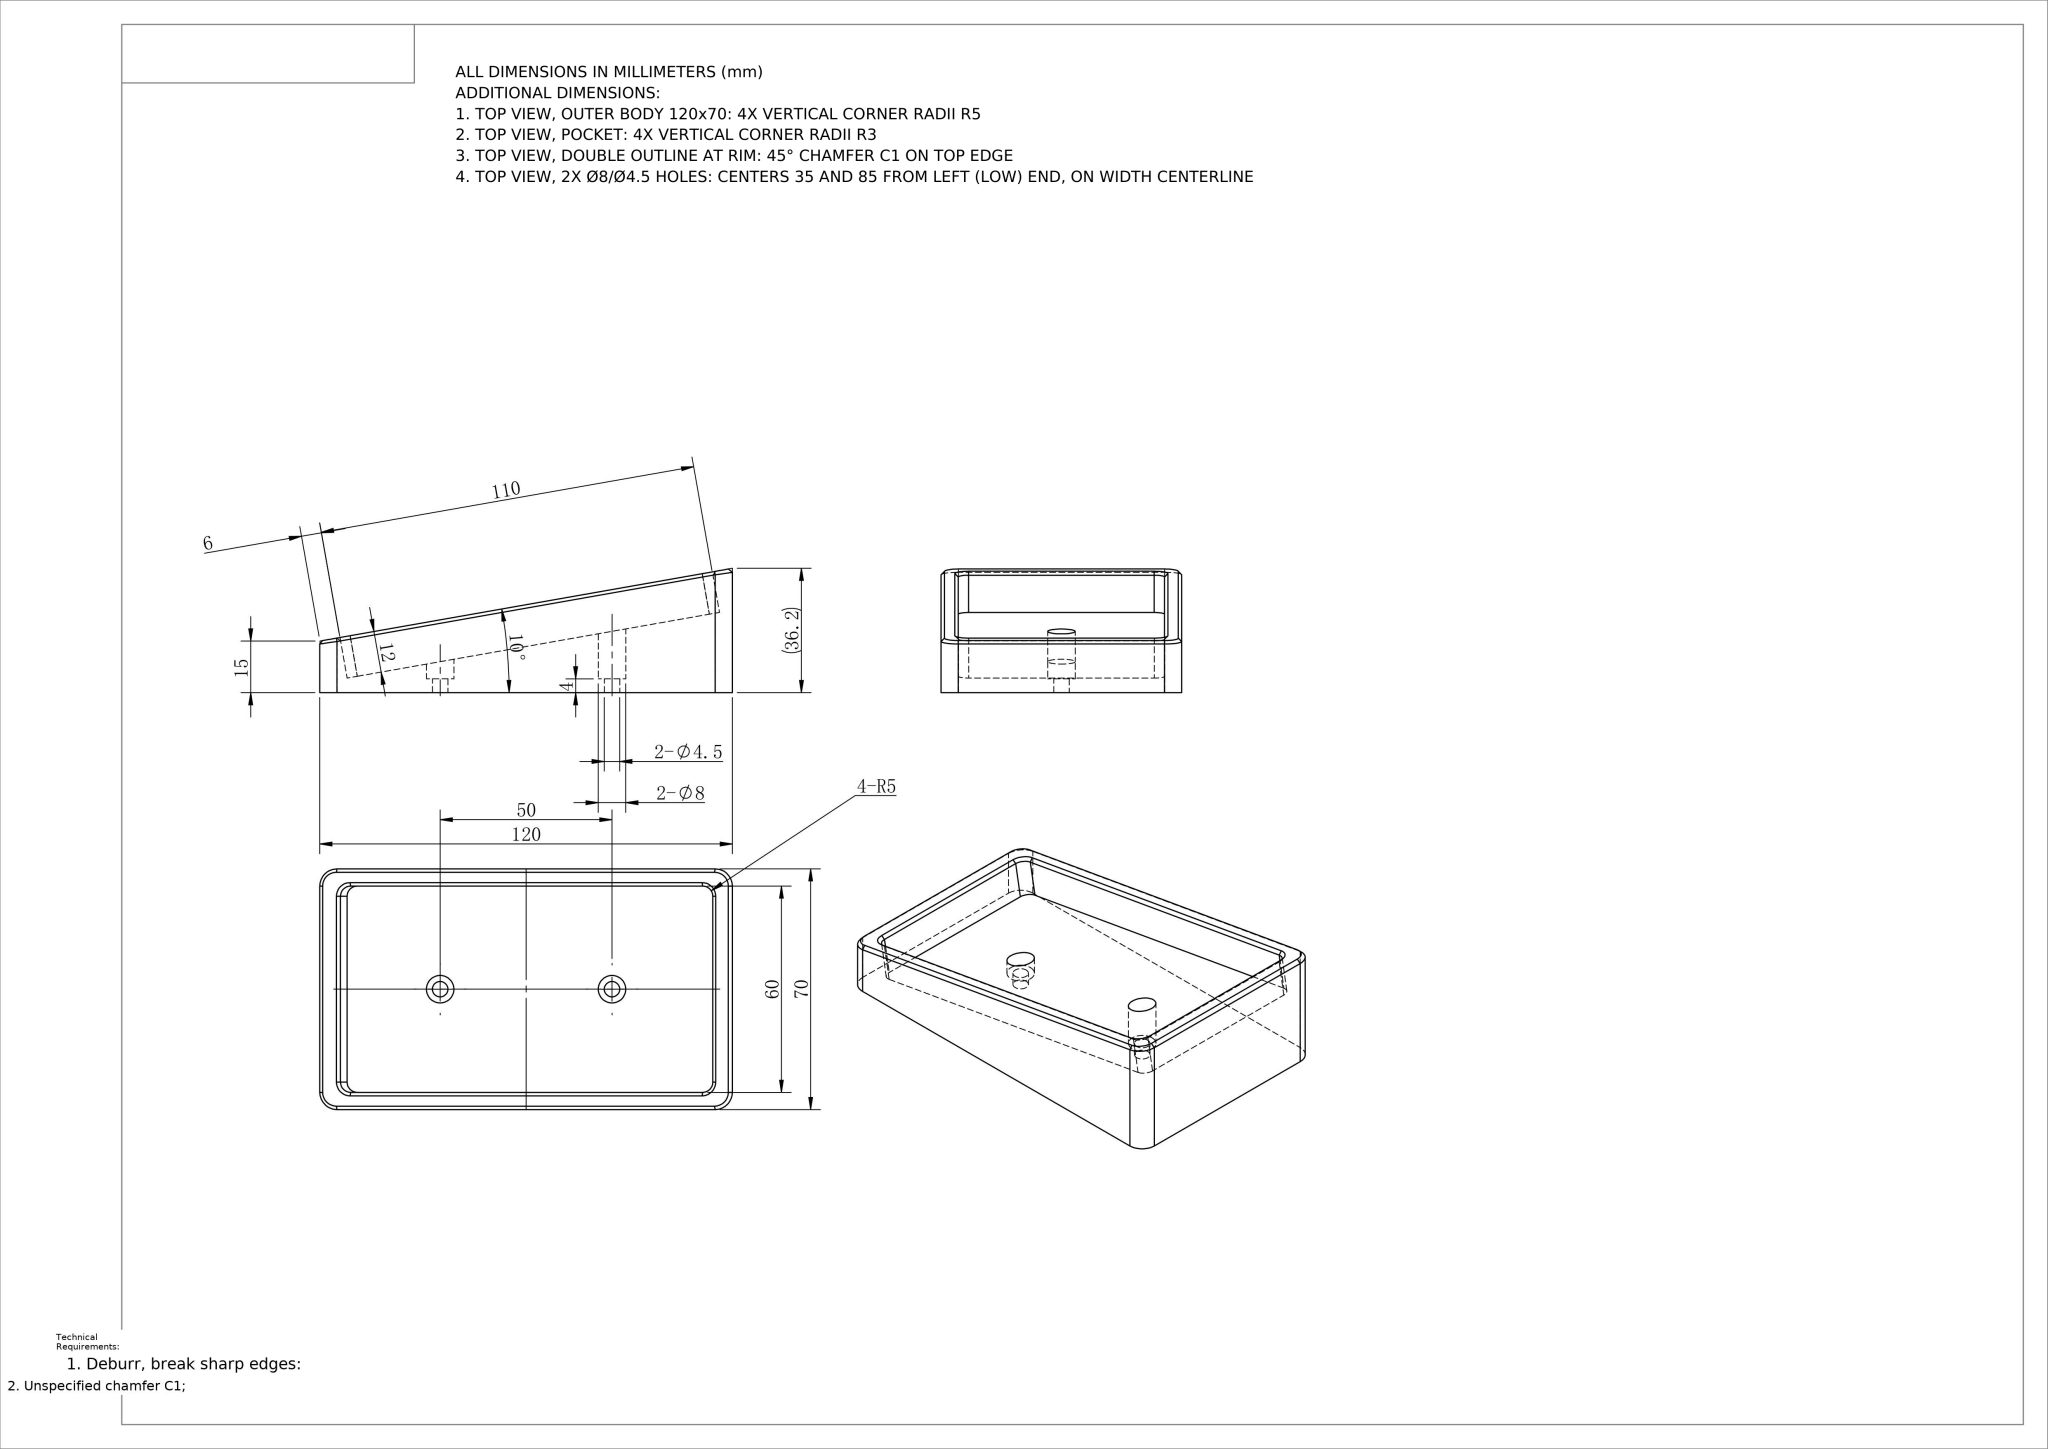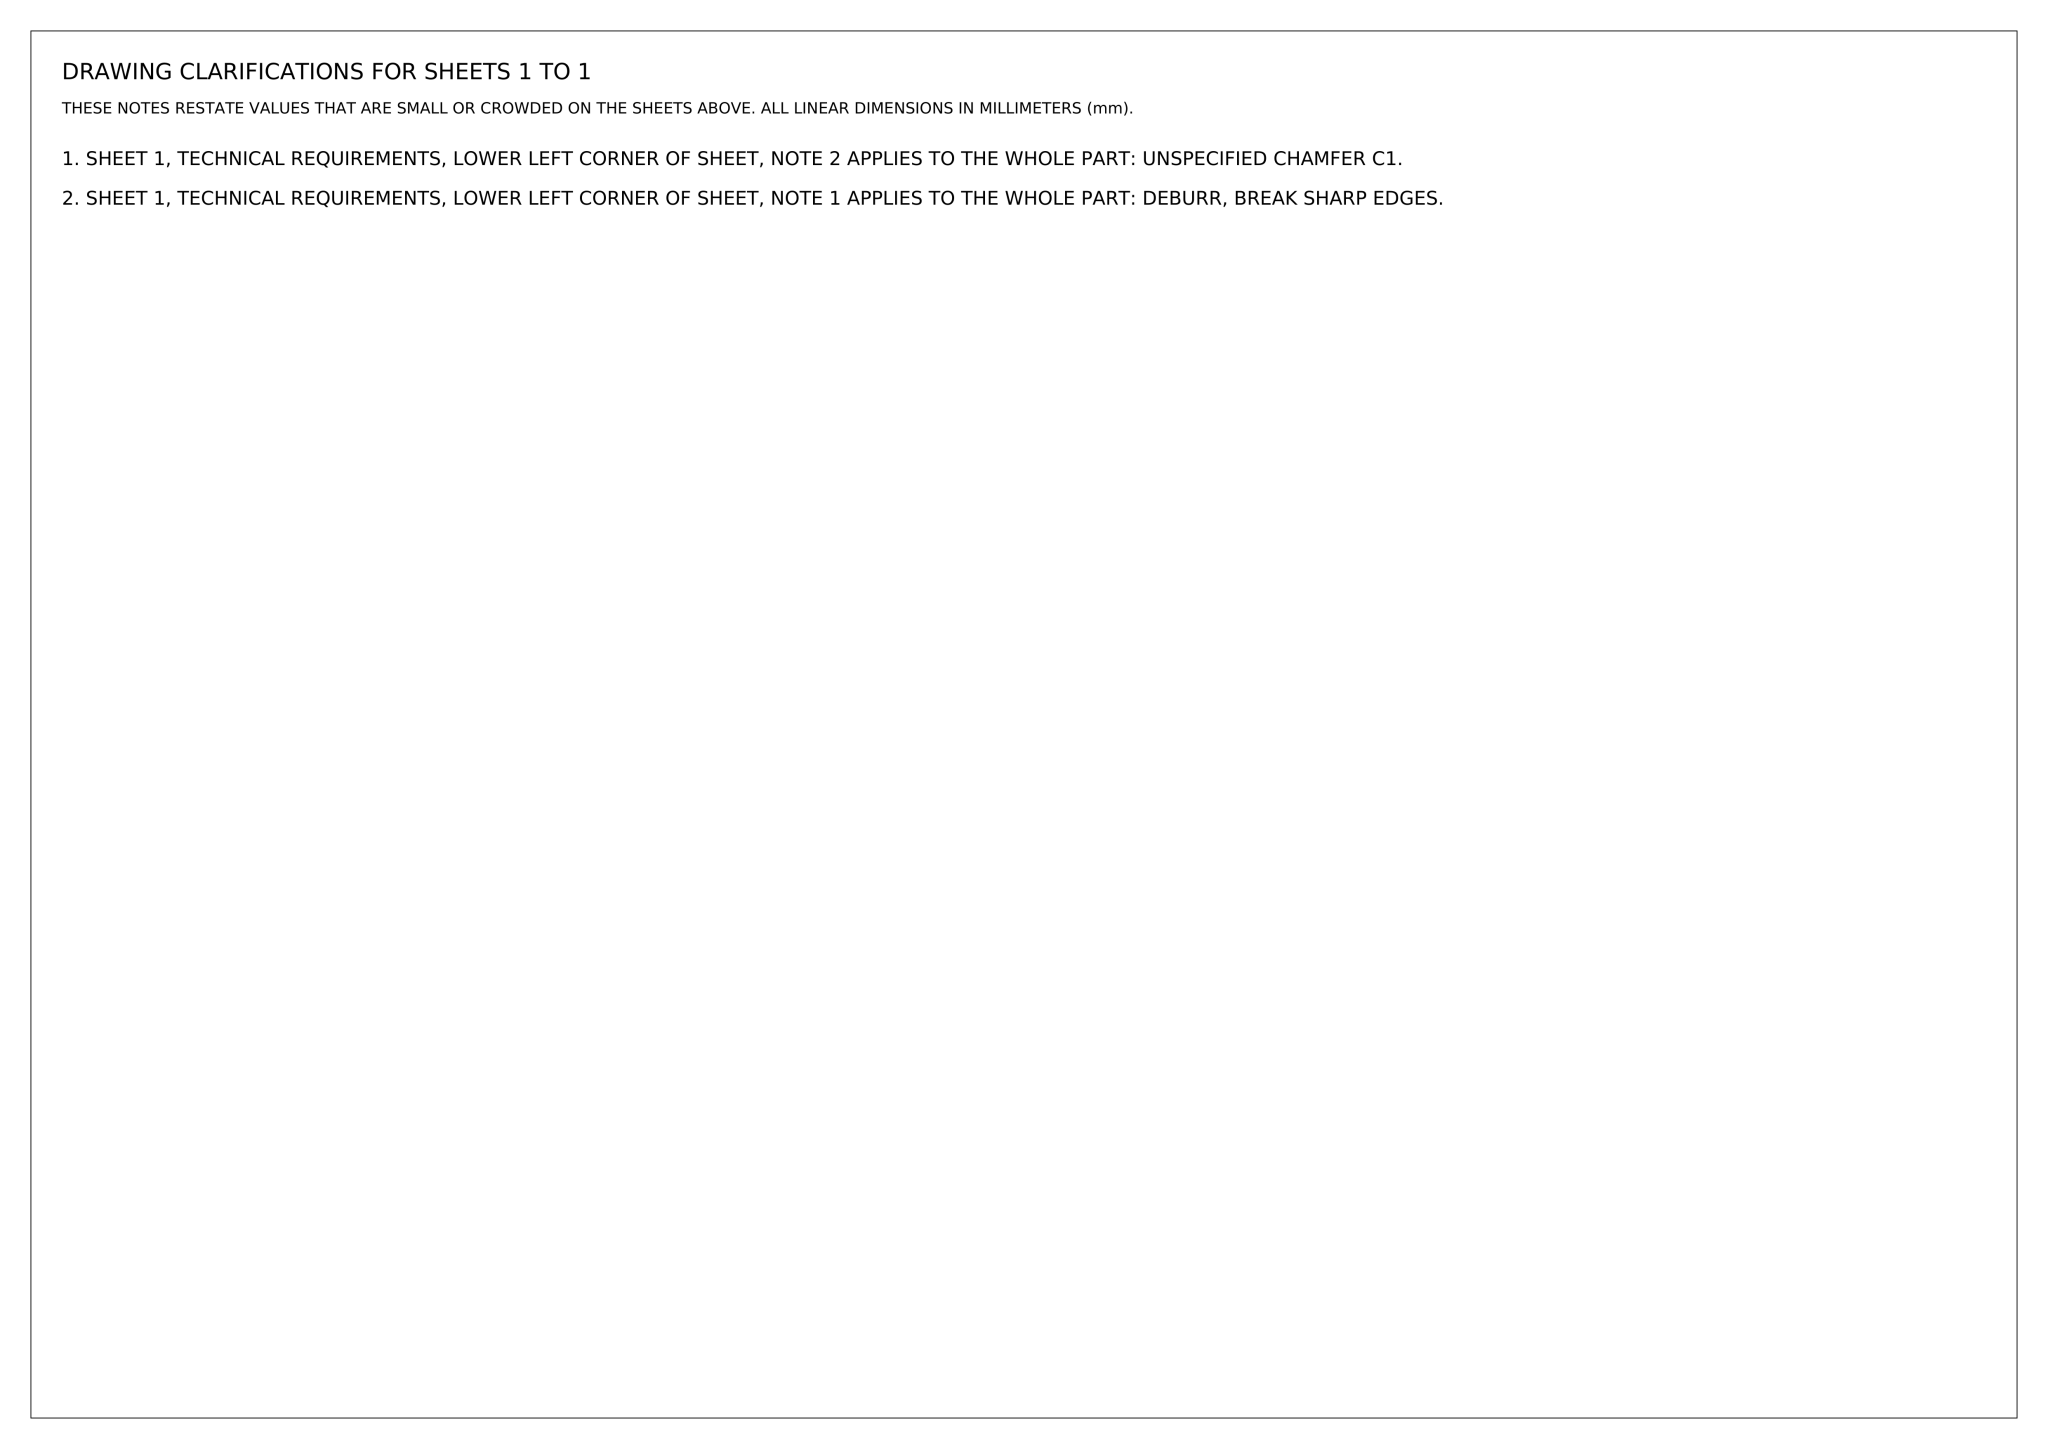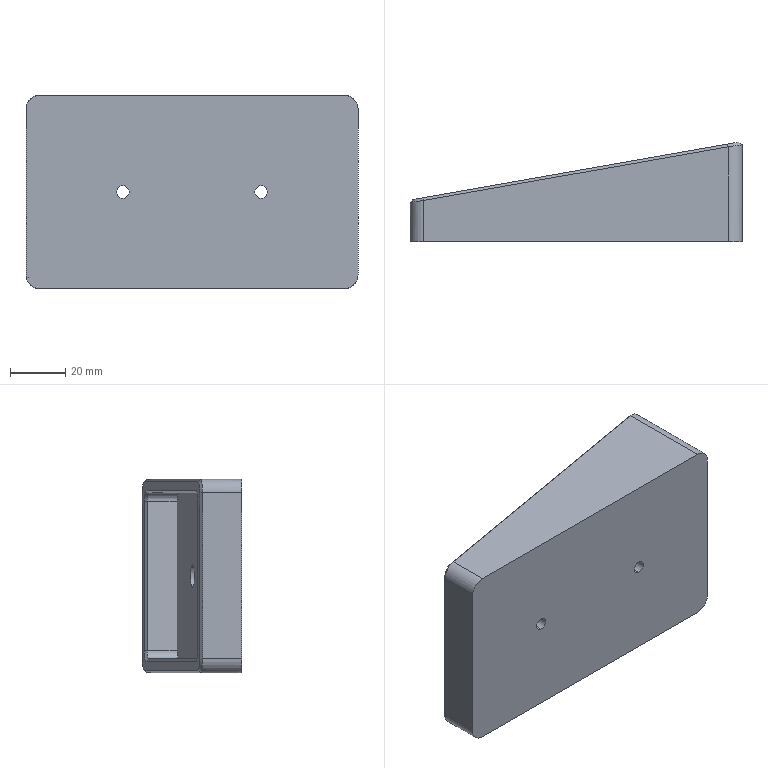Part | NX | mm | 1 solid | 45 faces | box 120 x 35.95 x 70 mm | volume 133782 mm3 | plane 21 | cylinder 16 | spline 4 | cone 4 | commonest cylinder face diameters 8 x4 4.5 x4 6 x4 10 x4